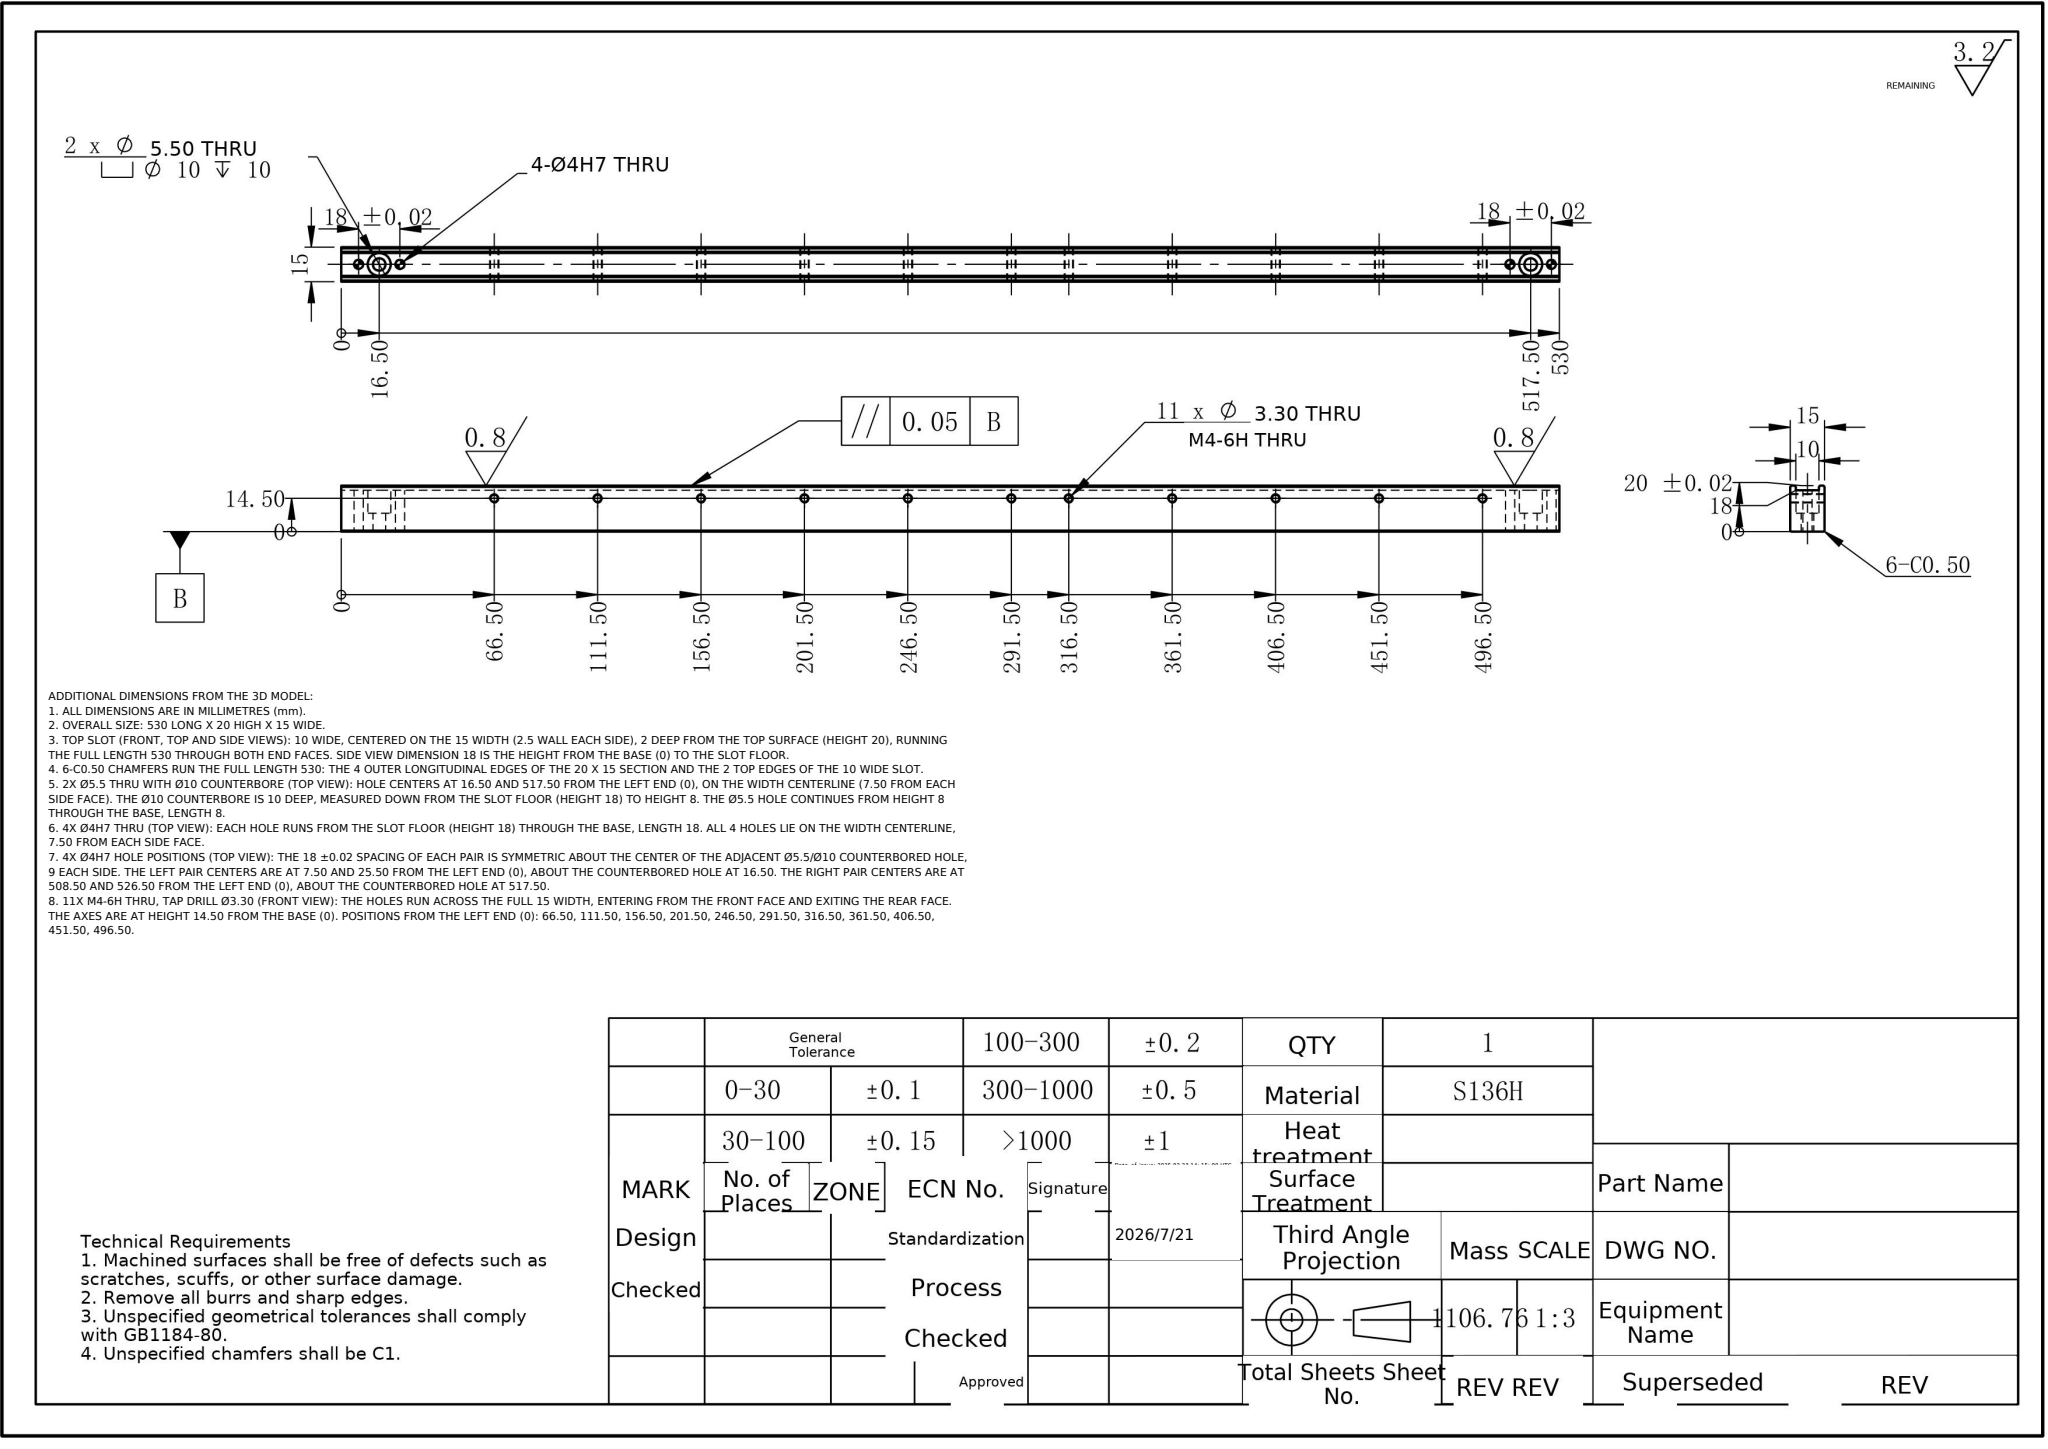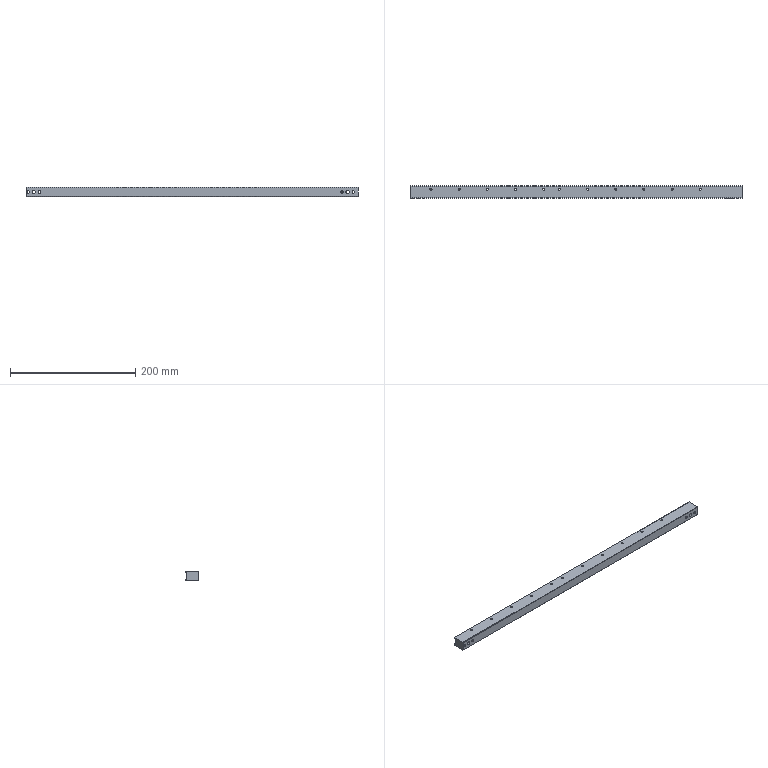Part | NX | mm | 1 solid | 58 faces | box 530 x 20 x 15 mm | volume 143736 mm3 | cylinder 38 | plane 20 | commonest cylinder face diameters 3.3 x22 4 x8 10 x4 5.5 x4